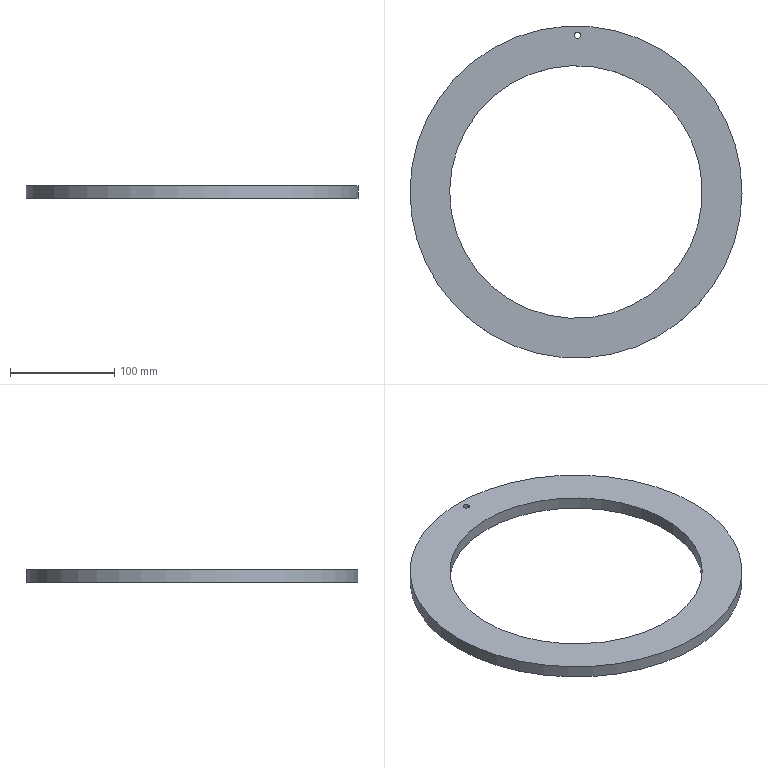Component | NX | FRICTION_DISC | 1 solid | 7 faces | box 318 x 318 x 12 mm | volume 400270 mm3 | cylinder 4 | plane 3 | commonest cylinder face diameters 318 x1 242 x1 6 x1 12 x1
STEP:
#1=CARTESIAN_POINT('',(0.,0.,0.));
#2=DIRECTION('',(0.,0.,1.));
#3=DIRECTION('',(1.,0.,0.));
#4=AXIS2_PLACEMENT_3D('',#1,#2,#3);
#5=CARTESIAN_POINT('',(-158.993,1.52,9.));
#6=VERTEX_POINT('',#5);
#7=CARTESIAN_POINT('',(0.,-0.,9.));
#8=DIRECTION('',(0.,0.,-1.));
#9=DIRECTION('',(-1.,0.009563,0.));
#10=AXIS2_PLACEMENT_3D('',#7,#8,#9);
#11=CIRCLE('',#10,159.);
#12=CARTESIAN_POINT('',(0.,-0.,9.));
#13=DIRECTION('',(0.,0.,1.));
#14=DIRECTION('',(1.,-0.009563,0.));
#15=AXIS2_PLACEMENT_3D('',#12,#13,#14);
#16=CYLINDRICAL_SURFACE('',#15,159.);
#17=CARTESIAN_POINT('',(9.425,0.));
#18=DIRECTION('',(-1.,0.));
#19=VECTOR('',#18,1.);
#20=LINE('',#17,#19);
#21=(GEOMETRIC_REPRESENTATION_CONTEXT(2)PARAMETRIC_REPRESENTATION_CONTEXT()REPRESENTATION_CONTEXT('',''));
#22=DEFINITIONAL_REPRESENTATION('',(#20),#21);
#23=PCURVE('',#16,#22);
#24=CARTESIAN_POINT('',(0.,-0.,9.));
#25=DIRECTION('',(0.,0.,-1.));
#26=DIRECTION('',(-1.,0.009563,0.));
#27=AXIS2_PLACEMENT_3D('',#24,#25,#26);
#28=PLANE('',#27);
#29=CARTESIAN_POINT('',(0.,0.));
#30=DIRECTION('',(1.,0.));
#31=AXIS2_PLACEMENT_2D('',#29,#30);
#32=CIRCLE('',#31,159.);
#33=(GEOMETRIC_REPRESENTATION_CONTEXT(2)PARAMETRIC_REPRESENTATION_CONTEXT()REPRESENTATION_CONTEXT('',''));
#34=DEFINITIONAL_REPRESENTATION('',(#32),#33);
#35=PCURVE('',#28,#34);
#36=SURFACE_CURVE('',#11,(#23,#35),.PCURVE_S1.);
#37=EDGE_CURVE('',#6,#6,#36,.T.);
#38=ORIENTED_EDGE('',*,*,#37,.F.);
#39=CARTESIAN_POINT('',(-158.993,1.52,21.));
#40=VERTEX_POINT('',#39);
#41=CARTESIAN_POINT('',(-158.993,1.52,9.));
#42=CARTESIAN_POINT('',(-158.993,1.52,21.));
#43=B_SPLINE_CURVE_WITH_KNOTS('',1,(#41,#42),.UNSPECIFIED.,.F.,.F.,(2,2),(0.,12.),.PIECEWISE_BEZIER_KNOTS.);
#44=CARTESIAN_POINT('',(9.425,0.));
#45=DIRECTION('',(0.,1.));
#46=VECTOR('',#45,1.);
#47=LINE('',#44,#46);
#48=(GEOMETRIC_REPRESENTATION_CONTEXT(2)PARAMETRIC_REPRESENTATION_CONTEXT()REPRESENTATION_CONTEXT('',''));
#49=DEFINITIONAL_REPRESENTATION('',(#47),#48);
#50=PCURVE('',#16,#49);
#51=CARTESIAN_POINT('',(3.142,0.));
#52=DIRECTION('',(0.,1.));
#53=VECTOR('',#52,1.);
#54=LINE('',#51,#53);
#55=(GEOMETRIC_REPRESENTATION_CONTEXT(2)PARAMETRIC_REPRESENTATION_CONTEXT()REPRESENTATION_CONTEXT('',''));
#56=DEFINITIONAL_REPRESENTATION('',(#54),#55);
#57=PCURVE('',#16,#56);
#58=SEAM_CURVE('',#43,(#50,#57),.PCURVE_S1.);
#59=EDGE_CURVE('',#6,#40,#58,.T.);
#60=ORIENTED_EDGE('',*,*,#59,.T.);
#61=CARTESIAN_POINT('',(0.,-0.,21.));
#62=DIRECTION('',(0.,0.,-1.));
#63=DIRECTION('',(-1.,0.009563,0.));
#64=AXIS2_PLACEMENT_3D('',#61,#62,#63);
#65=CIRCLE('',#64,159.);
#66=CARTESIAN_POINT('',(9.425,12.));
#67=DIRECTION('',(-1.,0.));
#68=VECTOR('',#67,1.);
#69=LINE('',#66,#68);
#70=(GEOMETRIC_REPRESENTATION_CONTEXT(2)PARAMETRIC_REPRESENTATION_CONTEXT()REPRESENTATION_CONTEXT('',''));
#71=DEFINITIONAL_REPRESENTATION('',(#69),#70);
#72=PCURVE('',#16,#71);
#73=CARTESIAN_POINT('',(0.,-0.,21.));
#74=DIRECTION('',(0.,0.,-1.));
#75=DIRECTION('',(-1.,0.009563,0.));
#76=AXIS2_PLACEMENT_3D('',#73,#74,#75);
#77=PLANE('',#76);
#78=CARTESIAN_POINT('',(0.,0.));
#79=DIRECTION('',(1.,0.));
#80=AXIS2_PLACEMENT_2D('',#78,#79);
#81=CIRCLE('',#80,159.);
#82=(GEOMETRIC_REPRESENTATION_CONTEXT(2)PARAMETRIC_REPRESENTATION_CONTEXT()REPRESENTATION_CONTEXT('',''));
#83=DEFINITIONAL_REPRESENTATION('',(#81),#82);
#84=PCURVE('',#77,#83);
#85=SURFACE_CURVE('',#65,(#72,#84),.PCURVE_S1.);
#86=EDGE_CURVE('',#40,#40,#85,.T.);
#87=ORIENTED_EDGE('',*,*,#86,.T.);
#88=ORIENTED_EDGE('',*,*,#59,.F.);
#89=EDGE_LOOP('',(#38,#60,#87,#88));
#90=FACE_BOUND('',#89,.T.);
#91=ADVANCED_FACE('',(#90),#16,.T.);
#92=CARTESIAN_POINT('',(-120.994,1.157,9.));
#93=VERTEX_POINT('',#92);
#94=CARTESIAN_POINT('',(0.,-0.,9.));
#95=DIRECTION('',(0.,0.,-1.));
#96=DIRECTION('',(-1.,0.009563,0.));
#97=AXIS2_PLACEMENT_3D('',#94,#95,#96);
#98=CIRCLE('',#97,121.);
#99=CARTESIAN_POINT('',(0.,-0.,9.));
#100=DIRECTION('',(0.,0.,1.));
#101=DIRECTION('',(1.,-0.009563,0.));
#102=AXIS2_PLACEMENT_3D('',#99,#100,#101);
#103=CYLINDRICAL_SURFACE('',#102,121.);
#104=CARTESIAN_POINT('',(9.425,0.));
#105=DIRECTION('',(-1.,0.));
#106=VECTOR('',#105,1.);
#107=LINE('',#104,#106);
#108=(GEOMETRIC_REPRESENTATION_CONTEXT(2)PARAMETRIC_REPRESENTATION_CONTEXT()REPRESENTATION_CONTEXT('',''));
#109=DEFINITIONAL_REPRESENTATION('',(#107),#108);
#110=PCURVE('',#103,#109);
#111=CARTESIAN_POINT('',(0.,0.));
#112=DIRECTION('',(1.,0.));
#113=AXIS2_PLACEMENT_2D('',#111,#112);
#114=CIRCLE('',#113,121.);
#115=(GEOMETRIC_REPRESENTATION_CONTEXT(2)PARAMETRIC_REPRESENTATION_CONTEXT()REPRESENTATION_CONTEXT('',''));
#116=DEFINITIONAL_REPRESENTATION('',(#114),#115);
#117=PCURVE('',#28,#116);
#118=SURFACE_CURVE('',#98,(#110,#117),.PCURVE_S1.);
#119=EDGE_CURVE('',#93,#93,#118,.T.);
#120=ORIENTED_EDGE('',*,*,#119,.F.);
#121=CARTESIAN_POINT('',(-120.994,1.157,21.));
#122=VERTEX_POINT('',#121);
#123=CARTESIAN_POINT('',(-120.994,1.157,9.));
#124=CARTESIAN_POINT('',(-120.994,1.157,21.));
#125=B_SPLINE_CURVE_WITH_KNOTS('',1,(#123,#124),.UNSPECIFIED.,.F.,.F.,(2,2),(0.,12.),.PIECEWISE_BEZIER_KNOTS.);
#126=CARTESIAN_POINT('',(9.425,0.));
#127=DIRECTION('',(0.,1.));
#128=VECTOR('',#127,1.);
#129=LINE('',#126,#128);
#130=(GEOMETRIC_REPRESENTATION_CONTEXT(2)PARAMETRIC_REPRESENTATION_CONTEXT()REPRESENTATION_CONTEXT('',''));
#131=DEFINITIONAL_REPRESENTATION('',(#129),#130);
#132=PCURVE('',#103,#131);
#133=CARTESIAN_POINT('',(3.142,0.));
#134=DIRECTION('',(0.,1.));
#135=VECTOR('',#134,1.);
#136=LINE('',#133,#135);
#137=(GEOMETRIC_REPRESENTATION_CONTEXT(2)PARAMETRIC_REPRESENTATION_CONTEXT()REPRESENTATION_CONTEXT('',''));
#138=DEFINITIONAL_REPRESENTATION('',(#136),#137);
#139=PCURVE('',#103,#138);
#140=SEAM_CURVE('',#125,(#132,#139),.PCURVE_S1.);
#141=EDGE_CURVE('',#93,#122,#140,.T.);
#142=ORIENTED_EDGE('',*,*,#141,.T.);
#143=CARTESIAN_POINT('',(0.,-0.,21.));
#144=DIRECTION('',(0.,0.,-1.));
#145=DIRECTION('',(-1.,0.009563,0.));
#146=AXIS2_PLACEMENT_3D('',#143,#144,#145);
#147=CIRCLE('',#146,121.);
#148=CARTESIAN_POINT('',(9.425,12.));
#149=DIRECTION('',(-1.,0.));
#150=VECTOR('',#149,1.);
#151=LINE('',#148,#150);
#152=(GEOMETRIC_REPRESENTATION_CONTEXT(2)PARAMETRIC_REPRESENTATION_CONTEXT()REPRESENTATION_CONTEXT('',''));
#153=DEFINITIONAL_REPRESENTATION('',(#151),#152);
#154=PCURVE('',#103,#153);
#155=CARTESIAN_POINT('',(0.,0.));
#156=DIRECTION('',(1.,0.));
#157=AXIS2_PLACEMENT_2D('',#155,#156);
#158=CIRCLE('',#157,121.);
#159=(GEOMETRIC_REPRESENTATION_CONTEXT(2)PARAMETRIC_REPRESENTATION_CONTEXT()REPRESENTATION_CONTEXT('',''));
#160=DEFINITIONAL_REPRESENTATION('',(#158),#159);
#161=PCURVE('',#77,#160);
#162=SURFACE_CURVE('',#147,(#154,#161),.PCURVE_S1.);
#163=EDGE_CURVE('',#122,#122,#162,.T.);
#164=ORIENTED_EDGE('',*,*,#163,.T.);
#165=ORIENTED_EDGE('',*,*,#141,.F.);
#166=EDGE_LOOP('',(#120,#142,#164,#165));
#167=FACE_BOUND('',#166,.F.);
#168=ADVANCED_FACE('',(#167),#103,.F.);
#169=CARTESIAN_POINT('',(7.434,149.936,9.));
#170=VERTEX_POINT('',#169);
#171=CARTESIAN_POINT('',(1.434,149.993,9.));
#172=DIRECTION('',(0.,0.,1.));
#173=DIRECTION('',(1.,-0.009563,0.));
#174=AXIS2_PLACEMENT_3D('',#171,#172,#173);
#175=CIRCLE('',#174,6.);
#176=CARTESIAN_POINT('',(-6.,150.));
#177=CARTESIAN_POINT('',(-6.,160.392));
#178=CARTESIAN_POINT('',(3.,155.196));
#179=CARTESIAN_POINT('',(12.,150.));
#180=CARTESIAN_POINT('',(3.,144.804));
#181=CARTESIAN_POINT('',(-6.,139.608));
#182=CARTESIAN_POINT('',(-6.,150.));
#183=(BOUNDED_CURVE()B_SPLINE_CURVE(2,(#176,#177,#178,#179,#180,#181,#182),.UNSPECIFIED.,.T.,.F.)B_SPLINE_CURVE_WITH_KNOTS((1,2,2,2,2,1),(-2.094,0.,2.094,4.189,6.283,8.378),.UNSPECIFIED.)CURVE()GEOMETRIC_REPRESENTATION_ITEM()RATIONAL_B_SPLINE_CURVE((1.,0.5,1.,0.5,1.,0.5,1.))REPRESENTATION_ITEM(''));
#184=(GEOMETRIC_REPRESENTATION_CONTEXT(2)PARAMETRIC_REPRESENTATION_CONTEXT()REPRESENTATION_CONTEXT('',''));
#185=DEFINITIONAL_REPRESENTATION('',(#183),#184);
#186=PCURVE('',#28,#185);
#187=CARTESIAN_POINT('',(1.434,149.993,9.));
#188=DIRECTION('',(0.,0.,1.));
#189=DIRECTION('',(1.,-0.009563,0.));
#190=AXIS2_PLACEMENT_3D('',#187,#188,#189);
#191=CYLINDRICAL_SURFACE('',#190,6.);
#192=CARTESIAN_POINT('',(0.,0.));
#193=DIRECTION('',(1.,0.));
#194=VECTOR('',#193,1.);
#195=LINE('',#192,#194);
#196=(GEOMETRIC_REPRESENTATION_CONTEXT(2)PARAMETRIC_REPRESENTATION_CONTEXT()REPRESENTATION_CONTEXT('',''));
#197=DEFINITIONAL_REPRESENTATION('',(#195),#196);
#198=PCURVE('',#191,#197);
#199=SURFACE_CURVE('',#175,(#186,#198),.PCURVE_S1.);
#200=EDGE_CURVE('',#170,#170,#199,.T.);
#201=ORIENTED_EDGE('',*,*,#200,.T.);
#202=EDGE_LOOP('',(#201));
#203=FACE_BOUND('',#202,.T.);
#204=ORIENTED_EDGE('',*,*,#37,.T.);
#205=EDGE_LOOP('',(#204));
#206=FACE_BOUND('',#205,.T.);
#207=ORIENTED_EDGE('',*,*,#119,.F.);
#208=EDGE_LOOP('',(#207));
#209=FACE_BOUND('',#208,.T.);
#210=ADVANCED_FACE('',(#203,#206,#209),#28,.T.);
#211=CARTESIAN_POINT('',(-1.565,150.022,21.));
#212=VERTEX_POINT('',#211);
#213=CARTESIAN_POINT('',(4.434,149.964,21.));
#214=VERTEX_POINT('',#213);
#215=CARTESIAN_POINT('',(1.434,149.993,21.));
#216=DIRECTION('',(0.,0.,-1.));
#217=DIRECTION('',(-1.,0.009563,0.));
#218=AXIS2_PLACEMENT_3D('',#215,#216,#217);
#219=CIRCLE('',#218,3.);
#220=CARTESIAN_POINT('',(-0.,150.));
#221=DIRECTION('',(1.,-0.));
#222=AXIS2_PLACEMENT_2D('',#220,#221);
#223=CIRCLE('',#222,3.);
#224=(GEOMETRIC_REPRESENTATION_CONTEXT(2)PARAMETRIC_REPRESENTATION_CONTEXT()REPRESENTATION_CONTEXT('',''));
#225=DEFINITIONAL_REPRESENTATION('',(#223),#224);
#226=PCURVE('',#77,#225);
#227=CARTESIAN_POINT('',(1.434,149.993,211.783));
#228=DIRECTION('',(0.,0.,1.));
#229=DIRECTION('',(1.,-0.009563,0.));
#230=AXIS2_PLACEMENT_3D('',#227,#228,#229);
#231=CYLINDRICAL_SURFACE('',#230,3.);
#232=CARTESIAN_POINT('',(3.142,-190.783));
#233=DIRECTION('',(-1.,0.));
#234=VECTOR('',#233,1.);
#235=LINE('',#232,#234);
#236=(GEOMETRIC_REPRESENTATION_CONTEXT(2)PARAMETRIC_REPRESENTATION_CONTEXT()REPRESENTATION_CONTEXT('',''));
#237=DEFINITIONAL_REPRESENTATION('',(#235),#236);
#238=PCURVE('',#231,#237);
#239=SURFACE_CURVE('',#219,(#226,#238),.PCURVE_S1.);
#240=EDGE_CURVE('',#212,#214,#239,.T.);
#241=ORIENTED_EDGE('',*,*,#240,.T.);
#242=CARTESIAN_POINT('',(1.434,149.993,21.));
#243=DIRECTION('',(0.,0.,-1.));
#244=DIRECTION('',(-1.,0.009563,0.));
#245=AXIS2_PLACEMENT_3D('',#242,#243,#244);
#246=CIRCLE('',#245,3.);
#247=CARTESIAN_POINT('',(-0.,150.));
#248=DIRECTION('',(1.,-0.));
#249=AXIS2_PLACEMENT_2D('',#247,#248);
#250=CIRCLE('',#249,3.);
#251=(GEOMETRIC_REPRESENTATION_CONTEXT(2)PARAMETRIC_REPRESENTATION_CONTEXT()REPRESENTATION_CONTEXT('',''));
#252=DEFINITIONAL_REPRESENTATION('',(#250),#251);
#253=PCURVE('',#77,#252);
#254=CARTESIAN_POINT('',(9.425,-190.783));
#255=DIRECTION('',(-1.,0.));
#256=VECTOR('',#255,1.);
#257=LINE('',#254,#256);
#258=(GEOMETRIC_REPRESENTATION_CONTEXT(2)PARAMETRIC_REPRESENTATION_CONTEXT()REPRESENTATION_CONTEXT('',''));
#259=DEFINITIONAL_REPRESENTATION('',(#257),#258);
#260=PCURVE('',#231,#259);
#261=SURFACE_CURVE('',#246,(#253,#260),.PCURVE_S1.);
#262=EDGE_CURVE('',#214,#212,#261,.T.);
#263=ORIENTED_EDGE('',*,*,#262,.T.);
#264=EDGE_LOOP('',(#241,#263));
#265=FACE_BOUND('',#264,.T.);
#266=ORIENTED_EDGE('',*,*,#86,.F.);
#267=EDGE_LOOP('',(#266));
#268=FACE_BOUND('',#267,.T.);
#269=ORIENTED_EDGE('',*,*,#163,.T.);
#270=EDGE_LOOP('',(#269));
#271=FACE_BOUND('',#270,.T.);
#272=ADVANCED_FACE('',(#265,#268,#271),#77,.F.);
#273=CARTESIAN_POINT('',(4.434,149.964,15.));
#274=VERTEX_POINT('',#273);
#275=CARTESIAN_POINT('',(1.434,149.993,15.));
#276=DIRECTION('',(0.,0.,1.));
#277=DIRECTION('',(1.,-0.009563,0.));
#278=AXIS2_PLACEMENT_3D('',#275,#276,#277);
#279=CIRCLE('',#278,3.);
#280=CARTESIAN_POINT('',(0.,-196.783));
#281=DIRECTION('',(1.,0.));
#282=VECTOR('',#281,1.);
#283=LINE('',#280,#282);
#284=(GEOMETRIC_REPRESENTATION_CONTEXT(2)PARAMETRIC_REPRESENTATION_CONTEXT()REPRESENTATION_CONTEXT('',''));
#285=DEFINITIONAL_REPRESENTATION('',(#283),#284);
#286=PCURVE('',#231,#285);
#287=CARTESIAN_POINT('',(1.434,149.993,15.));
#288=DIRECTION('',(0.,0.,1.));
#289=DIRECTION('',(1.,-0.009563,0.));
#290=AXIS2_PLACEMENT_3D('',#287,#288,#289);
#291=PLANE('',#290);
#292=CARTESIAN_POINT('',(0.,0.));
#293=DIRECTION('',(1.,0.));
#294=AXIS2_PLACEMENT_2D('',#292,#293);
#295=CIRCLE('',#294,3.);
#296=(GEOMETRIC_REPRESENTATION_CONTEXT(2)PARAMETRIC_REPRESENTATION_CONTEXT()REPRESENTATION_CONTEXT('',''));
#297=DEFINITIONAL_REPRESENTATION('',(#295),#296);
#298=PCURVE('',#291,#297);
#299=SURFACE_CURVE('',#279,(#286,#298),.PCURVE_S1.);
#300=EDGE_CURVE('',#274,#274,#299,.T.);
#301=ORIENTED_EDGE('',*,*,#300,.T.);
#302=CARTESIAN_POINT('',(4.434,149.964,15.));
#303=CARTESIAN_POINT('',(4.434,149.964,21.));
#304=B_SPLINE_CURVE_WITH_KNOTS('',1,(#302,#303),.UNSPECIFIED.,.F.,.F.,(2,2),(-196.783,-190.783),.PIECEWISE_BEZIER_KNOTS.);
#305=CARTESIAN_POINT('',(6.283,0.));
#306=DIRECTION('',(0.,1.));
#307=VECTOR('',#306,1.);
#308=LINE('',#305,#307);
#309=(GEOMETRIC_REPRESENTATION_CONTEXT(2)PARAMETRIC_REPRESENTATION_CONTEXT()REPRESENTATION_CONTEXT('',''));
#310=DEFINITIONAL_REPRESENTATION('',(#308),#309);
#311=PCURVE('',#231,#310);
#312=CARTESIAN_POINT('',(0.,0.));
#313=DIRECTION('',(0.,1.));
#314=VECTOR('',#313,1.);
#315=LINE('',#312,#314);
#316=(GEOMETRIC_REPRESENTATION_CONTEXT(2)PARAMETRIC_REPRESENTATION_CONTEXT()REPRESENTATION_CONTEXT('',''));
#317=DEFINITIONAL_REPRESENTATION('',(#315),#316);
#318=PCURVE('',#231,#317);
#319=SEAM_CURVE('',#304,(#311,#318),.PCURVE_S1.);
#320=EDGE_CURVE('',#274,#214,#319,.T.);
#321=ORIENTED_EDGE('',*,*,#320,.T.);
#322=ORIENTED_EDGE('',*,*,#262,.T.);
#323=ORIENTED_EDGE('',*,*,#240,.T.);
#324=ORIENTED_EDGE('',*,*,#320,.F.);
#325=EDGE_LOOP('',(#301,#321,#322,#323,#324));
#326=FACE_BOUND('',#325,.F.);
#327=ADVANCED_FACE('',(#326),#231,.F.);
#328=ORIENTED_EDGE('',*,*,#300,.T.);
#329=EDGE_LOOP('',(#328));
#330=FACE_BOUND('',#329,.T.);
#331=CARTESIAN_POINT('',(7.434,149.936,15.));
#332=VERTEX_POINT('',#331);
#333=CARTESIAN_POINT('',(1.434,149.993,15.));
#334=DIRECTION('',(0.,0.,1.));
#335=DIRECTION('',(1.,-0.009563,0.));
#336=AXIS2_PLACEMENT_3D('',#333,#334,#335);
#337=CIRCLE('',#336,6.);
#338=CARTESIAN_POINT('',(0.,0.));
#339=DIRECTION('',(1.,0.));
#340=AXIS2_PLACEMENT_2D('',#338,#339);
#341=CIRCLE('',#340,6.);
#342=(GEOMETRIC_REPRESENTATION_CONTEXT(2)PARAMETRIC_REPRESENTATION_CONTEXT()REPRESENTATION_CONTEXT('',''));
#343=DEFINITIONAL_REPRESENTATION('',(#341),#342);
#344=PCURVE('',#291,#343);
#345=CARTESIAN_POINT('',(0.,6.));
#346=DIRECTION('',(1.,0.));
#347=VECTOR('',#346,1.);
#348=LINE('',#345,#347);
#349=(GEOMETRIC_REPRESENTATION_CONTEXT(2)PARAMETRIC_REPRESENTATION_CONTEXT()REPRESENTATION_CONTEXT('',''));
#350=DEFINITIONAL_REPRESENTATION('',(#348),#349);
#351=PCURVE('',#191,#350);
#352=SURFACE_CURVE('',#337,(#344,#351),.PCURVE_S1.);
#353=EDGE_CURVE('',#332,#332,#352,.T.);
#354=ORIENTED_EDGE('',*,*,#353,.F.);
#355=EDGE_LOOP('',(#354));
#356=FACE_BOUND('',#355,.T.);
#357=ADVANCED_FACE('',(#330,#356),#291,.F.);
#358=ORIENTED_EDGE('',*,*,#353,.F.);
#359=CARTESIAN_POINT('',(7.434,149.936,9.));
#360=CARTESIAN_POINT('',(7.434,149.936,15.));
#361=B_SPLINE_CURVE_WITH_KNOTS('',1,(#359,#360),.UNSPECIFIED.,.F.,.F.,(2,2),(0.,6.),.PIECEWISE_BEZIER_KNOTS.);
#362=CARTESIAN_POINT('',(0.,0.));
#363=DIRECTION('',(0.,1.));
#364=VECTOR('',#363,1.);
#365=LINE('',#362,#364);
#366=(GEOMETRIC_REPRESENTATION_CONTEXT(2)PARAMETRIC_REPRESENTATION_CONTEXT()REPRESENTATION_CONTEXT('',''));
#367=DEFINITIONAL_REPRESENTATION('',(#365),#366);
#368=PCURVE('',#191,#367);
#369=CARTESIAN_POINT('',(6.283,0.));
#370=DIRECTION('',(0.,1.));
#371=VECTOR('',#370,1.);
#372=LINE('',#369,#371);
#373=(GEOMETRIC_REPRESENTATION_CONTEXT(2)PARAMETRIC_REPRESENTATION_CONTEXT()REPRESENTATION_CONTEXT('',''));
#374=DEFINITIONAL_REPRESENTATION('',(#372),#373);
#375=PCURVE('',#191,#374);
#376=SEAM_CURVE('',#361,(#368,#375),.PCURVE_S1.);
#377=EDGE_CURVE('',#170,#332,#376,.T.);
#378=ORIENTED_EDGE('',*,*,#377,.F.);
#379=ORIENTED_EDGE('',*,*,#200,.T.);
#380=ORIENTED_EDGE('',*,*,#377,.T.);
#381=EDGE_LOOP('',(#358,#378,#379,#380));
#382=FACE_BOUND('',#381,.F.);
#383=ADVANCED_FACE('',(#382),#191,.F.);
#384=CLOSED_SHELL('',(#91,#168,#210,#272,#327,#357,#383));
#385=MANIFOLD_SOLID_BREP('',#384);
#386=(LENGTH_UNIT()NAMED_UNIT(*)SI_UNIT(.MILLI.,.METRE.));
#387=UNCERTAINTY_MEASURE_WITH_UNIT(LENGTH_MEASURE(0.000005),#386,'','');
#388=(NAMED_UNIT(*)PLANE_ANGLE_UNIT()SI_UNIT($,.RADIAN.));
#389=(NAMED_UNIT(*)SI_UNIT($,.STERADIAN.)SOLID_ANGLE_UNIT());
#390=(GEOMETRIC_REPRESENTATION_CONTEXT(3)GLOBAL_UNCERTAINTY_ASSIGNED_CONTEXT((#387))GLOBAL_UNIT_ASSIGNED_CONTEXT((#386,#388,#389))REPRESENTATION_CONTEXT('',''));
#391=ADVANCED_BREP_SHAPE_REPRESENTATION('',(#4,#385),#390);